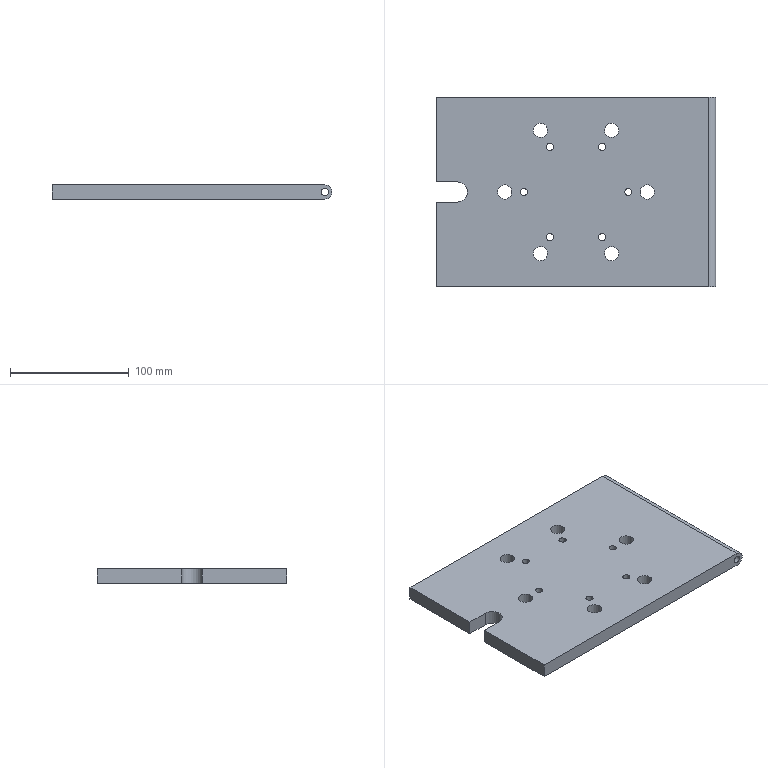Component | NX | DRILL_TEMPLATE | 1 solid | 23 faces | volume 430911 mm3 | cylinder 15 | plane 8 | commonest cylinder face diameters 12 x7 6 x7 17 x1